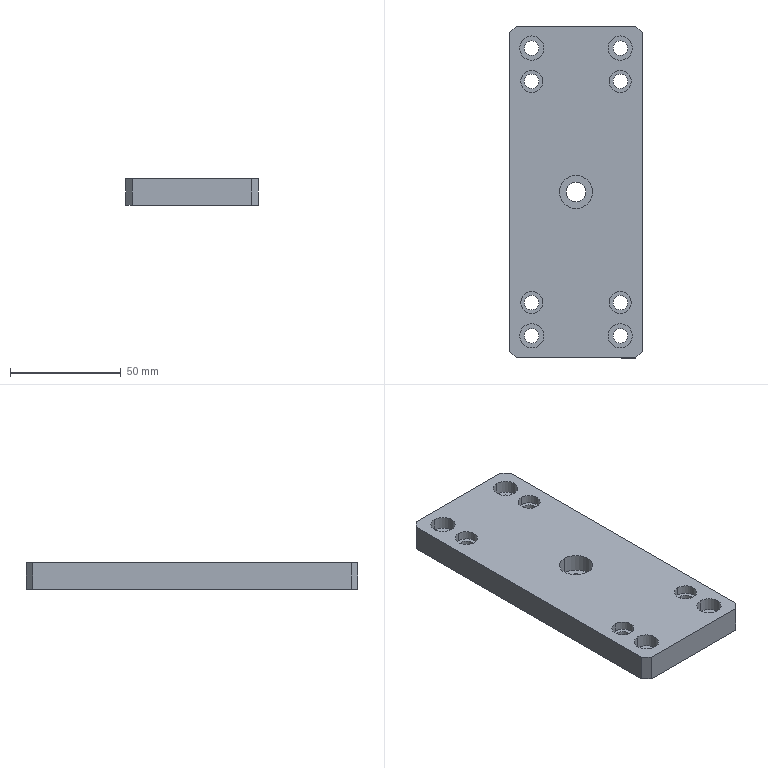Component | SolidWorks | A-C15UpperSupportPlate-1 | 1 solid | 79 faces | box 60 x 150 x 12 mm | volume 98743 mm3 | cylinder 52 | plane 27 | commonest cylinder face diameters 11 x16 6.6 x16 10 x8 12 x8 15 x2 9 x2
build123d program:
from build123d import *

# Parameters (mm, degrees)
SKETCH1_W                                       = 150
SKETCH1_H                                       = 60
EXTRUDE1_DEPTH                                  = 12
M6_HEX_SOCKET_HEAD_CAP_SCREW_CBORE1_D           = 6.6
M6_HEX_SOCKET_HEAD_CAP_SCREW_CBORE1_CBORE_D     = 11
M6_HEX_SOCKET_HEAD_CAP_SCREW_CBORE1_CBORE_DEPTH = 6
SKETCH4_R                                       = 6
EXTRUDE2_DEPTH                                  = 3
CHAMFER1_SIZE                                   = 3
SKETCH6_R                                       = 5
CUT_EXTRUDE1_DEPTH                              = 4
M6_HEX_SOCKET_HEAD_CAP_SCREW_CBORE2_D           = 6.6
M6_HEX_SOCKET_HEAD_CAP_SCREW_CBORE2_CBORE_D     = 11
M6_HEX_SOCKET_HEAD_CAP_SCREW_CBORE2_CBORE_DEPTH = 4
M8_HEX_SOCKET_HEAD_CAP_SCREW_CBORE1_D           = 9
M8_HEX_SOCKET_HEAD_CAP_SCREW_CBORE1_CBORE_D     = 15
M8_HEX_SOCKET_HEAD_CAP_SCREW_CBORE1_CBORE_DEPTH = 8


with BuildPart() as part:
    # Sketch1 → Extrude1 (new body)
    with BuildSketch(Plane.XY):
        Rectangle(SKETCH1_W, SKETCH1_H)
    extrude(amount=EXTRUDE1_DEPTH)

    # M6 Hex Socket Head Cap Screw CBORE1 (through all)
    with Locations(Plane.XY.offset(12)):
        with Locations((65, 20), (-65, 20), (-65, -20), (65, -20)):
            CounterBoreHole(M6_HEX_SOCKET_HEAD_CAP_SCREW_CBORE1_D / 2, M6_HEX_SOCKET_HEAD_CAP_SCREW_CBORE1_CBORE_D / 2, M6_HEX_SOCKET_HEAD_CAP_SCREW_CBORE1_CBORE_DEPTH)

    # Sketch4 → Extrude2 (cut)
    with BuildSketch(Plane(origin=(0, 0, 0), x_dir=(-1, 0, 0), z_dir=(0, 0, -1))):
        with Locations((-65, 20)):
            Circle(SKETCH4_R)
        with Locations((65, 20)):
            Circle(SKETCH4_R)
        with Locations((65, -20)):
            Circle(SKETCH4_R)
        with Locations((-65, -20)):
            Circle(SKETCH4_R)
    extrude(amount=-EXTRUDE2_DEPTH, mode=Mode.SUBTRACT)

    # Chamfer1
    chamfer1_edges = [part.edges().sort_by_distance(p)[0] for p in [
        (-75, 30, 6),
        (75, 30, 6),
        (75, -30, 6),
        (-75, -30, 6),
    ]]
    chamfer(chamfer1_edges, length=CHAMFER1_SIZE)

    # Sketch6 → Cut-Extrude1 (cut)
    with BuildSketch(Plane.XY.offset(12)):
        with Locations((-50, 20)):
            Circle(SKETCH6_R)
        with Locations((-50, -20)):
            Circle(SKETCH6_R)
        with Locations((50, 20)):
            Circle(SKETCH6_R)
        with Locations((50, -20)):
            Circle(SKETCH6_R)
    extrude(amount=-CUT_EXTRUDE1_DEPTH, mode=Mode.SUBTRACT)

    # M6 Hex Socket Head Cap Screw CBORE2 (through all)
    with Locations(Plane(origin=(0, 0, 0), x_dir=(-1, 0, 0), z_dir=(0, 0, -1))):
        with Locations((50, -20), (50, 20), (-50, -20), (-50, 20)):
            CounterBoreHole(M6_HEX_SOCKET_HEAD_CAP_SCREW_CBORE2_D / 2, M6_HEX_SOCKET_HEAD_CAP_SCREW_CBORE2_CBORE_D / 2, M6_HEX_SOCKET_HEAD_CAP_SCREW_CBORE2_CBORE_DEPTH)

    # M8 Hex Socket Head Cap Screw CBORE1 (through all)
    with Locations(Plane.XY.offset(12)):
        with Locations((0, 0)):
            CounterBoreHole(M8_HEX_SOCKET_HEAD_CAP_SCREW_CBORE1_D / 2, M8_HEX_SOCKET_HEAD_CAP_SCREW_CBORE1_CBORE_D / 2, M8_HEX_SOCKET_HEAD_CAP_SCREW_CBORE1_CBORE_DEPTH)


solid = part.part

# Placed as in the assembly
solid = solid.moved(Location((-33.181, 22.568, 15), (0, 0, 90)))